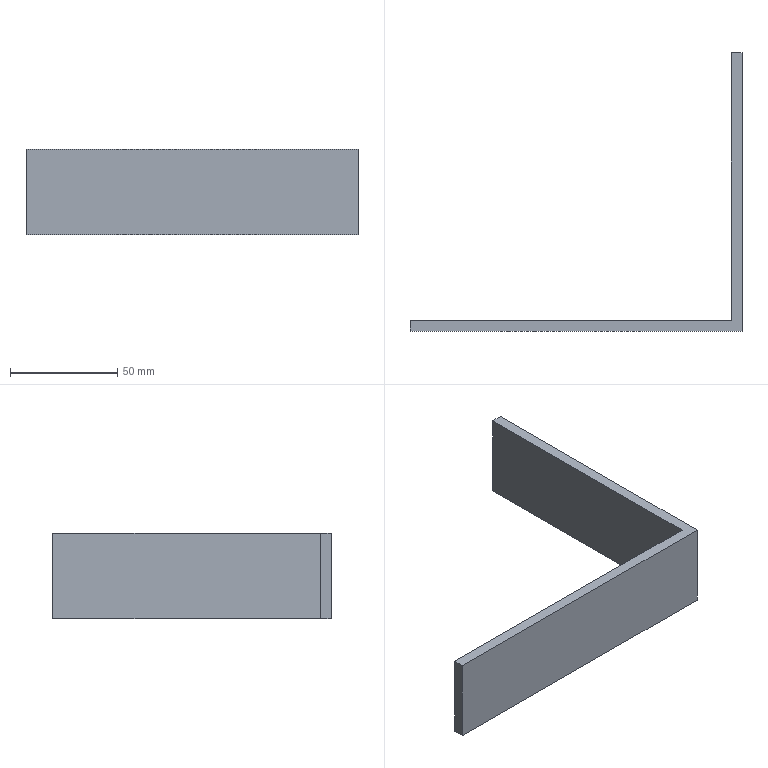Component | SolidWorks | SensorHolder-1 | 1 solid | 8 faces | box 155 x 130 x 40 mm | volume 56000 mm3 | plane 8 | material 45
build123d program:
from build123d import *

# Parameters (mm, degrees)
BOSS_EXTRUDE1_DEPTH = 40


with BuildPart() as part:
    # Sketch1 → Boss-Extrude1 (new body)
    with BuildSketch(Plane.XY):
        Polygon((0, 0), (150, 0), (150, 125), (155, 125), (155, -5), (0, -5), align=None)
    extrude(amount=BOSS_EXTRUDE1_DEPTH)


solid = part.part

# Placed as in the assembly
solid = solid.moved(Location((-391.359, -447.185, 1042), (0, 0, 0)))
STEP:
#1=CARTESIAN_POINT('',(-15.408,-17.606,41.024));
#2=VERTEX_POINT('',#1);
#3=CARTESIAN_POINT('',(-15.408,-17.803,41.024));
#4=VERTEX_POINT('',#3);
#5=CARTESIAN_POINT('',(-15.408,-17.803,41.024));
#6=DIRECTION('',(0.,-1.,0.));
#7=VECTOR('',#6,39.37);
#8=LINE('',#5,#7);
#9=EDGE_CURVE('',#2,#4,#8,.T.);
#10=ORIENTED_EDGE('',*,*,#9,.T.);
#11=CARTESIAN_POINT('',(-15.408,-17.803,42.598));
#12=VERTEX_POINT('',#11);
#13=CARTESIAN_POINT('',(-15.408,-17.803,42.598));
#14=DIRECTION('',(0.,0.,-1.));
#15=VECTOR('',#14,39.37);
#16=LINE('',#13,#15);
#17=EDGE_CURVE('',#12,#4,#16,.T.);
#18=ORIENTED_EDGE('',*,*,#17,.F.);
#19=CARTESIAN_POINT('',(-15.408,-17.606,42.598));
#20=VERTEX_POINT('',#19);
#21=CARTESIAN_POINT('',(-15.408,-17.803,42.598));
#22=DIRECTION('',(0.,-1.,0.));
#23=VECTOR('',#22,39.37);
#24=LINE('',#21,#23);
#25=EDGE_CURVE('',#20,#12,#24,.T.);
#26=ORIENTED_EDGE('',*,*,#25,.F.);
#27=CARTESIAN_POINT('',(-15.408,-17.606,42.598));
#28=DIRECTION('',(0.,0.,-1.));
#29=VECTOR('',#28,39.37);
#30=LINE('',#27,#29);
#31=EDGE_CURVE('',#20,#2,#30,.T.);
#32=ORIENTED_EDGE('',*,*,#31,.T.);
#33=EDGE_LOOP('',(#10,#18,#26,#32));
#34=FACE_OUTER_BOUND('',#33,.T.);
#35=CARTESIAN_POINT('',(-15.408,-17.803,42.598));
#36=DIRECTION('',(1.,0.,0.));
#37=DIRECTION('',(0.,0.,-1.));
#38=AXIS2_PLACEMENT_3D('',#35,#36,#37);
#39=PLANE('',#38);
#40=ADVANCED_FACE('',(#34),#39,.F.);
#41=CARTESIAN_POINT('',(-9.305,-17.803,41.024));
#42=VERTEX_POINT('',#41);
#43=CARTESIAN_POINT('',(-9.305,-17.803,41.024));
#44=DIRECTION('',(1.,0.,0.));
#45=VECTOR('',#44,39.37);
#46=LINE('',#43,#45);
#47=EDGE_CURVE('',#4,#42,#46,.T.);
#48=ORIENTED_EDGE('',*,*,#47,.T.);
#49=CARTESIAN_POINT('',(-9.305,-17.803,42.598));
#50=VERTEX_POINT('',#49);
#51=CARTESIAN_POINT('',(-9.305,-17.803,42.598));
#52=DIRECTION('',(0.,0.,-1.));
#53=VECTOR('',#52,39.37);
#54=LINE('',#51,#53);
#55=EDGE_CURVE('',#50,#42,#54,.T.);
#56=ORIENTED_EDGE('',*,*,#55,.F.);
#57=CARTESIAN_POINT('',(-9.305,-17.803,42.598));
#58=DIRECTION('',(1.,0.,0.));
#59=VECTOR('',#58,39.37);
#60=LINE('',#57,#59);
#61=EDGE_CURVE('',#12,#50,#60,.T.);
#62=ORIENTED_EDGE('',*,*,#61,.F.);
#63=ORIENTED_EDGE('',*,*,#17,.T.);
#64=EDGE_LOOP('',(#48,#56,#62,#63));
#65=FACE_OUTER_BOUND('',#64,.T.);
#66=CARTESIAN_POINT('',(-9.305,-17.803,42.598));
#67=DIRECTION('',(-0.,1.,0.));
#68=DIRECTION('',(-1.,-0.,0.));
#69=AXIS2_PLACEMENT_3D('',#66,#67,#68);
#70=PLANE('',#69);
#71=ADVANCED_FACE('',(#65),#70,.F.);
#72=CARTESIAN_POINT('',(-9.305,-12.684,41.024));
#73=VERTEX_POINT('',#72);
#74=CARTESIAN_POINT('',(-9.305,-12.684,41.024));
#75=DIRECTION('',(0.,1.,0.));
#76=VECTOR('',#75,39.37);
#77=LINE('',#74,#76);
#78=EDGE_CURVE('',#42,#73,#77,.T.);
#79=ORIENTED_EDGE('',*,*,#78,.T.);
#80=CARTESIAN_POINT('',(-9.305,-12.684,42.598));
#81=VERTEX_POINT('',#80);
#82=CARTESIAN_POINT('',(-9.305,-12.684,42.598));
#83=DIRECTION('',(0.,0.,-1.));
#84=VECTOR('',#83,39.37);
#85=LINE('',#82,#84);
#86=EDGE_CURVE('',#81,#73,#85,.T.);
#87=ORIENTED_EDGE('',*,*,#86,.F.);
#88=CARTESIAN_POINT('',(-9.305,-12.684,42.598));
#89=DIRECTION('',(0.,1.,0.));
#90=VECTOR('',#89,39.37);
#91=LINE('',#88,#90);
#92=EDGE_CURVE('',#50,#81,#91,.T.);
#93=ORIENTED_EDGE('',*,*,#92,.F.);
#94=ORIENTED_EDGE('',*,*,#55,.T.);
#95=EDGE_LOOP('',(#79,#87,#93,#94));
#96=FACE_OUTER_BOUND('',#95,.T.);
#97=CARTESIAN_POINT('',(-9.305,-12.684,42.598));
#98=DIRECTION('',(-1.,0.,0.));
#99=DIRECTION('',(0.,0.,1.));
#100=AXIS2_PLACEMENT_3D('',#97,#98,#99);
#101=PLANE('',#100);
#102=ADVANCED_FACE('',(#96),#101,.F.);
#103=CARTESIAN_POINT('',(-9.502,-12.684,41.024));
#104=VERTEX_POINT('',#103);
#105=CARTESIAN_POINT('',(-9.502,-12.684,41.024));
#106=DIRECTION('',(-1.,0.,0.));
#107=VECTOR('',#106,39.37);
#108=LINE('',#105,#107);
#109=EDGE_CURVE('',#73,#104,#108,.T.);
#110=ORIENTED_EDGE('',*,*,#109,.T.);
#111=CARTESIAN_POINT('',(-9.502,-12.684,42.598));
#112=VERTEX_POINT('',#111);
#113=CARTESIAN_POINT('',(-9.502,-12.684,42.598));
#114=DIRECTION('',(0.,0.,-1.));
#115=VECTOR('',#114,39.37);
#116=LINE('',#113,#115);
#117=EDGE_CURVE('',#112,#104,#116,.T.);
#118=ORIENTED_EDGE('',*,*,#117,.F.);
#119=CARTESIAN_POINT('',(-9.502,-12.684,42.598));
#120=DIRECTION('',(-1.,0.,0.));
#121=VECTOR('',#120,39.37);
#122=LINE('',#119,#121);
#123=EDGE_CURVE('',#81,#112,#122,.T.);
#124=ORIENTED_EDGE('',*,*,#123,.F.);
#125=ORIENTED_EDGE('',*,*,#86,.T.);
#126=EDGE_LOOP('',(#110,#118,#124,#125));
#127=FACE_OUTER_BOUND('',#126,.T.);
#128=CARTESIAN_POINT('',(-9.502,-12.684,42.598));
#129=DIRECTION('',(0.,-1.,0.));
#130=DIRECTION('',(0.,0.,-1.));
#131=AXIS2_PLACEMENT_3D('',#128,#129,#130);
#132=PLANE('',#131);
#133=ADVANCED_FACE('',(#127),#132,.F.);
#134=CARTESIAN_POINT('',(-9.502,-17.606,41.024));
#135=VERTEX_POINT('',#134);
#136=CARTESIAN_POINT('',(-9.502,-17.606,41.024));
#137=DIRECTION('',(0.,-1.,0.));
#138=VECTOR('',#137,39.37);
#139=LINE('',#136,#138);
#140=EDGE_CURVE('',#104,#135,#139,.T.);
#141=ORIENTED_EDGE('',*,*,#140,.T.);
#142=CARTESIAN_POINT('',(-9.502,-17.606,42.598));
#143=VERTEX_POINT('',#142);
#144=CARTESIAN_POINT('',(-9.502,-17.606,42.598));
#145=DIRECTION('',(0.,0.,-1.));
#146=VECTOR('',#145,39.37);
#147=LINE('',#144,#146);
#148=EDGE_CURVE('',#143,#135,#147,.T.);
#149=ORIENTED_EDGE('',*,*,#148,.F.);
#150=CARTESIAN_POINT('',(-9.502,-17.606,42.598));
#151=DIRECTION('',(0.,-1.,0.));
#152=VECTOR('',#151,39.37);
#153=LINE('',#150,#152);
#154=EDGE_CURVE('',#112,#143,#153,.T.);
#155=ORIENTED_EDGE('',*,*,#154,.F.);
#156=ORIENTED_EDGE('',*,*,#117,.T.);
#157=EDGE_LOOP('',(#141,#149,#155,#156));
#158=FACE_OUTER_BOUND('',#157,.T.);
#159=CARTESIAN_POINT('',(-9.502,-17.606,42.598));
#160=DIRECTION('',(1.,0.,0.));
#161=DIRECTION('',(0.,0.,-1.));
#162=AXIS2_PLACEMENT_3D('',#159,#160,#161);
#163=PLANE('',#162);
#164=ADVANCED_FACE('',(#158),#163,.F.);
#165=CARTESIAN_POINT('',(-15.408,-17.606,41.024));
#166=DIRECTION('',(-1.,0.,0.));
#167=VECTOR('',#166,39.37);
#168=LINE('',#165,#167);
#169=EDGE_CURVE('',#135,#2,#168,.T.);
#170=ORIENTED_EDGE('',*,*,#169,.T.);
#171=ORIENTED_EDGE('',*,*,#31,.F.);
#172=CARTESIAN_POINT('',(-15.408,-17.606,42.598));
#173=DIRECTION('',(-1.,0.,0.));
#174=VECTOR('',#173,39.37);
#175=LINE('',#172,#174);
#176=EDGE_CURVE('',#143,#20,#175,.T.);
#177=ORIENTED_EDGE('',*,*,#176,.F.);
#178=ORIENTED_EDGE('',*,*,#148,.T.);
#179=EDGE_LOOP('',(#170,#171,#177,#178));
#180=FACE_OUTER_BOUND('',#179,.T.);
#181=CARTESIAN_POINT('',(-15.408,-17.606,42.598));
#182=DIRECTION('',(0.,-1.,0.));
#183=DIRECTION('',(0.,0.,-1.));
#184=AXIS2_PLACEMENT_3D('',#181,#182,#183);
#185=PLANE('',#184);
#186=ADVANCED_FACE('',(#180),#185,.F.);
#187=ORIENTED_EDGE('',*,*,#25,.T.);
#188=ORIENTED_EDGE('',*,*,#61,.T.);
#189=ORIENTED_EDGE('',*,*,#92,.T.);
#190=ORIENTED_EDGE('',*,*,#123,.T.);
#191=ORIENTED_EDGE('',*,*,#154,.T.);
#192=ORIENTED_EDGE('',*,*,#176,.T.);
#193=EDGE_LOOP('',(#187,#188,#189,#190,#191,#192));
#194=FACE_OUTER_BOUND('',#193,.T.);
#195=CARTESIAN_POINT('',(-15.408,-17.606,42.598));
#196=DIRECTION('',(0.,0.,-1.));
#197=DIRECTION('',(-1.,0.,0.));
#198=AXIS2_PLACEMENT_3D('',#195,#196,#197);
#199=PLANE('',#198);
#200=ADVANCED_FACE('',(#194),#199,.F.);
#201=ORIENTED_EDGE('',*,*,#9,.F.);
#202=ORIENTED_EDGE('',*,*,#169,.F.);
#203=ORIENTED_EDGE('',*,*,#140,.F.);
#204=ORIENTED_EDGE('',*,*,#109,.F.);
#205=ORIENTED_EDGE('',*,*,#78,.F.);
#206=ORIENTED_EDGE('',*,*,#47,.F.);
#207=EDGE_LOOP('',(#201,#202,#203,#204,#205,#206));
#208=FACE_OUTER_BOUND('',#207,.T.);
#209=CARTESIAN_POINT('',(-15.408,-17.606,41.024));
#210=DIRECTION('',(0.,0.,-1.));
#211=DIRECTION('',(-1.,0.,0.));
#212=AXIS2_PLACEMENT_3D('',#209,#210,#211);
#213=PLANE('',#212);
#214=ADVANCED_FACE('',(#208),#213,.T.);
#215=CLOSED_SHELL('',(#40,#71,#102,#133,#164,#186,#200,#214));
#216=MANIFOLD_SOLID_BREP('',#215);
#217=CARTESIAN_POINT('',(0.,0.,0.));
#218=DIRECTION('',(0.,0.,1.));
#219=DIRECTION('',(1.,0.,0.));
#220=AXIS2_PLACEMENT_3D('',#217,#218,#219);
#221=(LENGTH_UNIT()NAMED_UNIT(*)SI_UNIT($,.METRE.));
#222=LENGTH_MEASURE_WITH_UNIT(LENGTH_MEASURE(0.0254),#221);
#223=DIMENSIONAL_EXPONENTS(1.,0.,0.,0.,0.,0.,0.);
#224=(CONVERSION_BASED_UNIT('',#222)LENGTH_UNIT()NAMED_UNIT(#223));
#225=UNCERTAINTY_MEASURE_WITH_UNIT(LENGTH_MEASURE(0.00001),#224,'','');
#226=(NAMED_UNIT(*)PLANE_ANGLE_UNIT()SI_UNIT($,.RADIAN.));
#227=(NAMED_UNIT(*)SI_UNIT($,.STERADIAN.)SOLID_ANGLE_UNIT());
#228=(GEOMETRIC_REPRESENTATION_CONTEXT(3)GLOBAL_UNCERTAINTY_ASSIGNED_CONTEXT((#225))GLOBAL_UNIT_ASSIGNED_CONTEXT((#224,#226,#227))REPRESENTATION_CONTEXT('',''));
#229=ADVANCED_BREP_SHAPE_REPRESENTATION('',(#216,#220),#228);
#230=COLOUR_RGB('',0.7922,0.8196,0.9333);
#231=FILL_AREA_STYLE_COLOUR('',#230);
#232=FILL_AREA_STYLE('',(#231));
#233=SURFACE_STYLE_FILL_AREA(#232);
#234=SURFACE_SIDE_STYLE('',(#233));
#235=SURFACE_STYLE_USAGE(.BOTH.,#234);
#236=PRESENTATION_STYLE_ASSIGNMENT((#235));
#237=STYLED_ITEM('',(#236),#216);
#238=PRESENTATION_LAYER_ASSIGNMENT('','',(#237));
#239=(LENGTH_UNIT()NAMED_UNIT(*)SI_UNIT($,.METRE.));
#240=LENGTH_MEASURE_WITH_UNIT(LENGTH_MEASURE(0.0254),#239);
#241=DIMENSIONAL_EXPONENTS(1.,0.,0.,0.,0.,0.,0.);
#242=(CONVERSION_BASED_UNIT('',#240)LENGTH_UNIT()NAMED_UNIT(#241));
#243=UNCERTAINTY_MEASURE_WITH_UNIT(LENGTH_MEASURE(0.00001),#242,'','');
#244=(NAMED_UNIT(*)PLANE_ANGLE_UNIT()SI_UNIT($,.RADIAN.));
#245=(NAMED_UNIT(*)SI_UNIT($,.STERADIAN.)SOLID_ANGLE_UNIT());
#246=(GEOMETRIC_REPRESENTATION_CONTEXT(3)GLOBAL_UNCERTAINTY_ASSIGNED_CONTEXT((#243))GLOBAL_UNIT_ASSIGNED_CONTEXT((#242,#244,#245))REPRESENTATION_CONTEXT('',''));
#247=MECHANICAL_DESIGN_GEOMETRIC_PRESENTATION_REPRESENTATION('',(#237),#246);